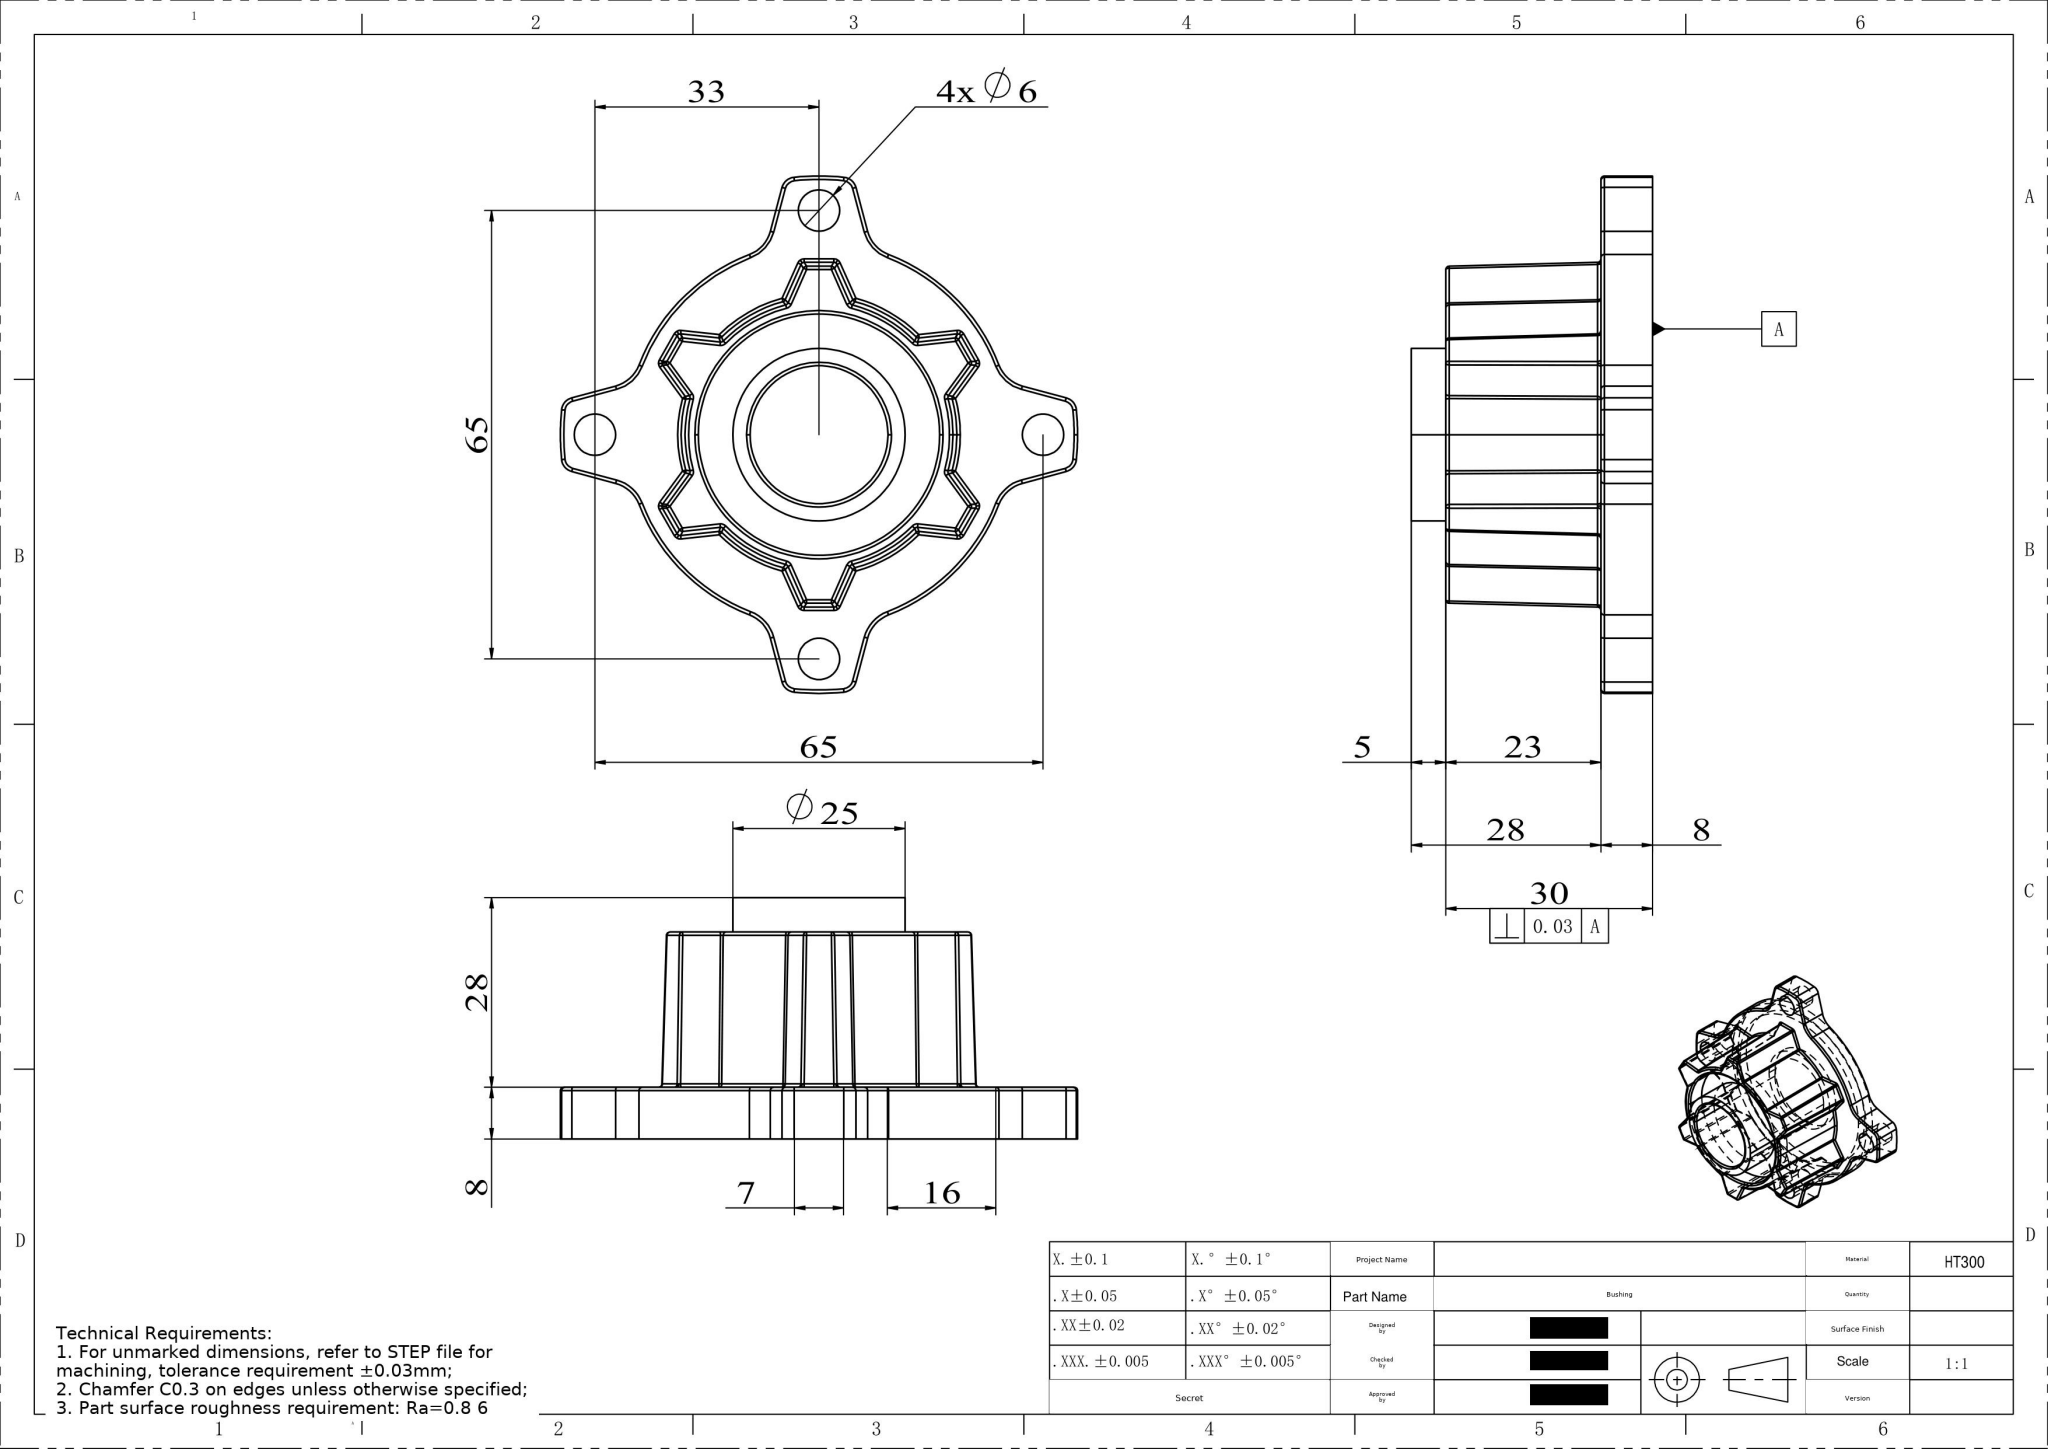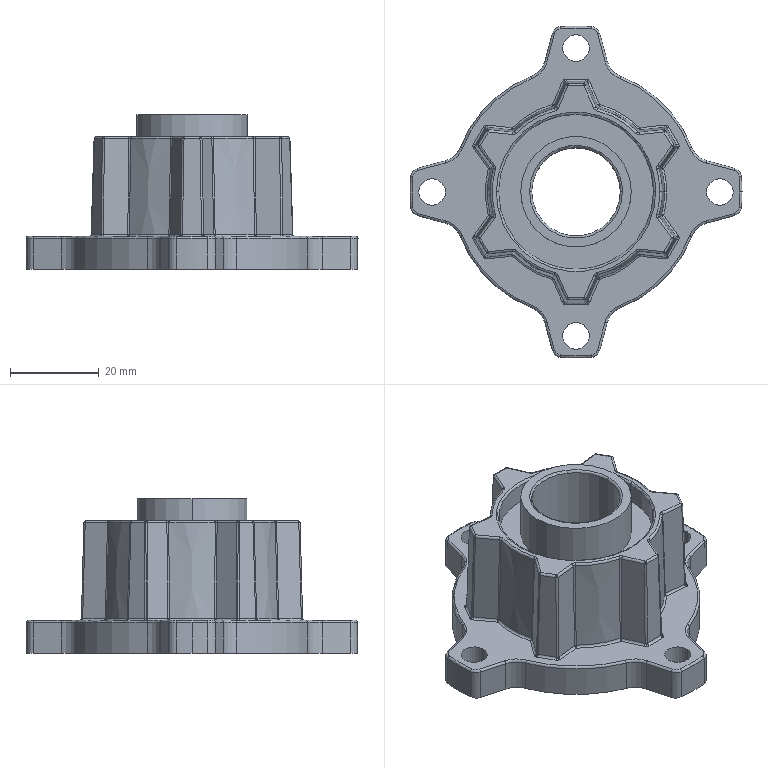Part | SolidWorks | mm | material HT300 | 1 solid | 289 faces | box 75 x 75 x 35 mm | volume 40949 mm3 | cylinder 105 | sphere 52 | spline 48 | torus 43 | plane 34 | cone 7 | commonest cylinder face diameters 1 x60 6 x8 10 x8 4 x8 75 x5 56 x4 20 x2 24.8 x2